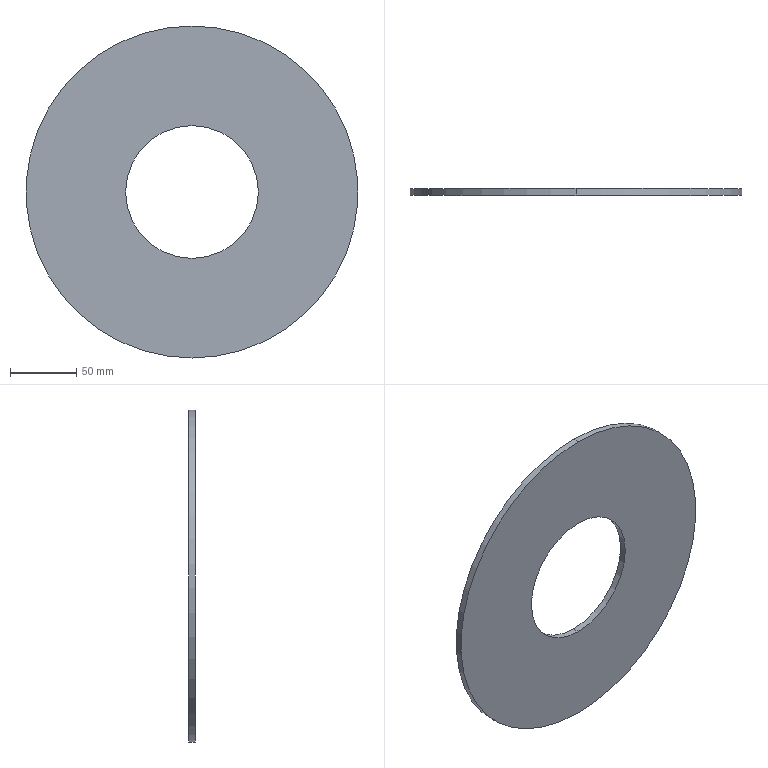Component | SolidWorks | Support2-2 | 1 solid | 6 faces | box 250 x 5 x 250 mm | volume 206167 mm3 | cylinder 4 | plane 2 | commonest cylinder face diameters 100 x2 250 x2 | material Plain Carbon Steel
STEP:
#1=COLOUR_RGB('',0.7922,0.8196,0.9333);
#2=FILL_AREA_STYLE_COLOUR('',#1);
#3=FILL_AREA_STYLE('',(#2));
#4=SURFACE_STYLE_FILL_AREA(#3);
#5=SURFACE_SIDE_STYLE('',(#4));
#6=SURFACE_STYLE_USAGE(.BOTH.,#5);
#7=PRESENTATION_STYLE_ASSIGNMENT((#6));
#8=CARTESIAN_POINT('',(49.235,57.14,70.988));
#9=VERTEX_POINT('',#8);
#10=CARTESIAN_POINT('',(49.235,57.14,74.925));
#11=VERTEX_POINT('',#10);
#12=CARTESIAN_POINT('',(49.235,57.14,72.956));
#13=DIRECTION('',(-0.,-1.,-0.));
#14=DIRECTION('',(0.,-0.,1.));
#15=AXIS2_PLACEMENT_3D('',#12,#13,#14);
#16=CIRCLE('',#15,1.969);
#17=EDGE_CURVE('',#9,#11,#16,.T.);
#18=ORIENTED_EDGE('',*,*,#17,.F.);
#19=CARTESIAN_POINT('',(49.235,56.943,70.988));
#20=VERTEX_POINT('',#19);
#21=CARTESIAN_POINT('',(49.235,57.14,70.988));
#22=DIRECTION('',(-0.,-1.,-0.));
#23=VECTOR('',#22,39.37);
#24=LINE('',#21,#23);
#25=EDGE_CURVE('',#9,#20,#24,.T.);
#26=ORIENTED_EDGE('',*,*,#25,.T.);
#27=CARTESIAN_POINT('',(49.235,56.943,74.925));
#28=VERTEX_POINT('',#27);
#29=CARTESIAN_POINT('',(49.235,56.943,72.956));
#30=DIRECTION('',(-0.,-1.,-0.));
#31=DIRECTION('',(0.,-0.,1.));
#32=AXIS2_PLACEMENT_3D('',#29,#30,#31);
#33=CIRCLE('',#32,1.969);
#34=EDGE_CURVE('',#20,#28,#33,.T.);
#35=ORIENTED_EDGE('',*,*,#34,.T.);
#36=CARTESIAN_POINT('',(49.235,57.14,74.925));
#37=DIRECTION('',(-0.,-1.,-0.));
#38=VECTOR('',#37,39.37);
#39=LINE('',#36,#38);
#40=EDGE_CURVE('',#11,#28,#39,.T.);
#41=ORIENTED_EDGE('',*,*,#40,.F.);
#42=EDGE_LOOP('',(#18,#26,#35,#41));
#43=FACE_OUTER_BOUND('',#42,.T.);
#44=CARTESIAN_POINT('',(49.235,57.14,72.956));
#45=DIRECTION('',(-0.,-1.,-0.));
#46=DIRECTION('',(0.,-0.,1.));
#47=AXIS2_PLACEMENT_3D('',#44,#45,#46);
#48=CYLINDRICAL_SURFACE('',#47,1.969);
#49=ADVANCED_FACE('',(#43),#48,.F.);
#50=CARTESIAN_POINT('',(49.235,57.14,77.877));
#51=VERTEX_POINT('',#50);
#52=CARTESIAN_POINT('',(49.235,57.14,68.035));
#53=VERTEX_POINT('',#52);
#54=CARTESIAN_POINT('',(49.235,57.14,72.956));
#55=DIRECTION('',(-0.,-1.,-0.));
#56=DIRECTION('',(0.,-0.,1.));
#57=AXIS2_PLACEMENT_3D('',#54,#55,#56);
#58=CIRCLE('',#57,4.921);
#59=EDGE_CURVE('',#51,#53,#58,.T.);
#60=ORIENTED_EDGE('',*,*,#59,.T.);
#61=CARTESIAN_POINT('',(49.235,56.943,68.035));
#62=VERTEX_POINT('',#61);
#63=CARTESIAN_POINT('',(49.235,57.14,68.035));
#64=DIRECTION('',(-0.,-1.,-0.));
#65=VECTOR('',#64,39.37);
#66=LINE('',#63,#65);
#67=EDGE_CURVE('',#53,#62,#66,.T.);
#68=ORIENTED_EDGE('',*,*,#67,.T.);
#69=CARTESIAN_POINT('',(49.235,56.943,77.877));
#70=VERTEX_POINT('',#69);
#71=CARTESIAN_POINT('',(49.235,56.943,72.956));
#72=DIRECTION('',(-0.,-1.,-0.));
#73=DIRECTION('',(0.,-0.,1.));
#74=AXIS2_PLACEMENT_3D('',#71,#72,#73);
#75=CIRCLE('',#74,4.921);
#76=EDGE_CURVE('',#70,#62,#75,.T.);
#77=ORIENTED_EDGE('',*,*,#76,.F.);
#78=CARTESIAN_POINT('',(49.235,57.14,77.877));
#79=DIRECTION('',(-0.,-1.,-0.));
#80=VECTOR('',#79,39.37);
#81=LINE('',#78,#80);
#82=EDGE_CURVE('',#51,#70,#81,.T.);
#83=ORIENTED_EDGE('',*,*,#82,.F.);
#84=EDGE_LOOP('',(#60,#68,#77,#83));
#85=FACE_OUTER_BOUND('',#84,.T.);
#86=CARTESIAN_POINT('',(49.235,57.14,72.956));
#87=DIRECTION('',(-0.,-1.,-0.));
#88=DIRECTION('',(0.,-0.,1.));
#89=AXIS2_PLACEMENT_3D('',#86,#87,#88);
#90=CYLINDRICAL_SURFACE('',#89,4.921);
#91=ADVANCED_FACE('',(#85),#90,.T.);
#92=ORIENTED_EDGE('',*,*,#67,.F.);
#93=CARTESIAN_POINT('',(49.235,57.14,72.956));
#94=DIRECTION('',(-0.,-1.,-0.));
#95=DIRECTION('',(0.,-0.,1.));
#96=AXIS2_PLACEMENT_3D('',#93,#94,#95);
#97=CIRCLE('',#96,4.921);
#98=EDGE_CURVE('',#53,#51,#97,.T.);
#99=ORIENTED_EDGE('',*,*,#98,.T.);
#100=ORIENTED_EDGE('',*,*,#82,.T.);
#101=CARTESIAN_POINT('',(49.235,56.943,72.956));
#102=DIRECTION('',(-0.,-1.,-0.));
#103=DIRECTION('',(0.,-0.,1.));
#104=AXIS2_PLACEMENT_3D('',#101,#102,#103);
#105=CIRCLE('',#104,4.921);
#106=EDGE_CURVE('',#62,#70,#105,.T.);
#107=ORIENTED_EDGE('',*,*,#106,.F.);
#108=EDGE_LOOP('',(#92,#99,#100,#107));
#109=FACE_OUTER_BOUND('',#108,.T.);
#110=CARTESIAN_POINT('',(49.235,57.14,72.956));
#111=DIRECTION('',(-0.,-1.,-0.));
#112=DIRECTION('',(0.,-0.,1.));
#113=AXIS2_PLACEMENT_3D('',#110,#111,#112);
#114=CYLINDRICAL_SURFACE('',#113,4.921);
#115=ADVANCED_FACE('',(#109),#114,.T.);
#116=CARTESIAN_POINT('',(49.235,57.14,72.956));
#117=DIRECTION('',(-0.,-1.,-0.));
#118=DIRECTION('',(0.,-0.,1.));
#119=AXIS2_PLACEMENT_3D('',#116,#117,#118);
#120=CIRCLE('',#119,1.969);
#121=EDGE_CURVE('',#11,#9,#120,.T.);
#122=ORIENTED_EDGE('',*,*,#121,.T.);
#123=ORIENTED_EDGE('',*,*,#17,.T.);
#124=EDGE_LOOP('',(#122,#123));
#125=FACE_BOUND('',#124,.T.);
#126=ORIENTED_EDGE('',*,*,#59,.F.);
#127=ORIENTED_EDGE('',*,*,#98,.F.);
#128=EDGE_LOOP('',(#126,#127));
#129=FACE_OUTER_BOUND('',#128,.T.);
#130=CARTESIAN_POINT('',(49.235,57.14,72.956));
#131=DIRECTION('',(-0.,-1.,-0.));
#132=DIRECTION('',(0.,-0.,1.));
#133=AXIS2_PLACEMENT_3D('',#130,#131,#132);
#134=PLANE('',#133);
#135=ADVANCED_FACE('',(#125,#129),#134,.F.);
#136=CARTESIAN_POINT('',(49.235,56.943,72.956));
#137=DIRECTION('',(-0.,-1.,-0.));
#138=DIRECTION('',(0.,-0.,1.));
#139=AXIS2_PLACEMENT_3D('',#136,#137,#138);
#140=CIRCLE('',#139,1.969);
#141=EDGE_CURVE('',#28,#20,#140,.T.);
#142=ORIENTED_EDGE('',*,*,#141,.F.);
#143=ORIENTED_EDGE('',*,*,#34,.F.);
#144=EDGE_LOOP('',(#142,#143));
#145=FACE_BOUND('',#144,.T.);
#146=ORIENTED_EDGE('',*,*,#76,.T.);
#147=ORIENTED_EDGE('',*,*,#106,.T.);
#148=EDGE_LOOP('',(#146,#147));
#149=FACE_OUTER_BOUND('',#148,.T.);
#150=CARTESIAN_POINT('',(49.235,56.943,72.956));
#151=DIRECTION('',(-0.,-1.,-0.));
#152=DIRECTION('',(0.,-0.,1.));
#153=AXIS2_PLACEMENT_3D('',#150,#151,#152);
#154=PLANE('',#153);
#155=ADVANCED_FACE('',(#145,#149),#154,.T.);
#156=ORIENTED_EDGE('',*,*,#25,.F.);
#157=ORIENTED_EDGE('',*,*,#121,.F.);
#158=ORIENTED_EDGE('',*,*,#40,.T.);
#159=ORIENTED_EDGE('',*,*,#141,.T.);
#160=EDGE_LOOP('',(#156,#157,#158,#159));
#161=FACE_OUTER_BOUND('',#160,.T.);
#162=CARTESIAN_POINT('',(49.235,57.14,72.956));
#163=DIRECTION('',(-0.,-1.,-0.));
#164=DIRECTION('',(0.,-0.,1.));
#165=AXIS2_PLACEMENT_3D('',#162,#163,#164);
#166=CYLINDRICAL_SURFACE('',#165,1.969);
#167=ADVANCED_FACE('',(#161),#166,.F.);
#168=CLOSED_SHELL('',(#49,#91,#115,#135,#155,#167));
#169=MANIFOLD_SOLID_BREP('',#168);
#170=STYLED_ITEM('',(#7),#169);
#171=PRESENTATION_LAYER_ASSIGNMENT('','',(#170));
#172=CARTESIAN_POINT('',(0.,0.,0.));
#173=DIRECTION('',(0.,0.,1.));
#174=DIRECTION('',(1.,0.,0.));
#175=AXIS2_PLACEMENT_3D('',#172,#173,#174);
#176=(LENGTH_UNIT()NAMED_UNIT(*)SI_UNIT($,.METRE.));
#177=LENGTH_MEASURE_WITH_UNIT(LENGTH_MEASURE(0.0254),#176);
#178=DIMENSIONAL_EXPONENTS(1.,0.,0.,0.,0.,0.,0.);
#179=(CONVERSION_BASED_UNIT('',#177)LENGTH_UNIT()NAMED_UNIT(#178));
#180=UNCERTAINTY_MEASURE_WITH_UNIT(LENGTH_MEASURE(0.00001),#179,'','');
#181=(NAMED_UNIT(*)PLANE_ANGLE_UNIT()SI_UNIT($,.RADIAN.));
#182=(NAMED_UNIT(*)SI_UNIT($,.STERADIAN.)SOLID_ANGLE_UNIT());
#183=(GEOMETRIC_REPRESENTATION_CONTEXT(3)GLOBAL_UNCERTAINTY_ASSIGNED_CONTEXT((#180))GLOBAL_UNIT_ASSIGNED_CONTEXT((#179,#181,#182))REPRESENTATION_CONTEXT('',''));
#184=ADVANCED_BREP_SHAPE_REPRESENTATION('',(#169,#175),#183);
#185=(LENGTH_UNIT()NAMED_UNIT(*)SI_UNIT($,.METRE.));
#186=LENGTH_MEASURE_WITH_UNIT(LENGTH_MEASURE(0.0254),#185);
#187=DIMENSIONAL_EXPONENTS(1.,0.,0.,0.,0.,0.,0.);
#188=(CONVERSION_BASED_UNIT('',#186)LENGTH_UNIT()NAMED_UNIT(#187));
#189=UNCERTAINTY_MEASURE_WITH_UNIT(LENGTH_MEASURE(0.00001),#188,'','');
#190=(NAMED_UNIT(*)PLANE_ANGLE_UNIT()SI_UNIT($,.RADIAN.));
#191=(NAMED_UNIT(*)SI_UNIT($,.STERADIAN.)SOLID_ANGLE_UNIT());
#192=(GEOMETRIC_REPRESENTATION_CONTEXT(3)GLOBAL_UNCERTAINTY_ASSIGNED_CONTEXT((#189))GLOBAL_UNIT_ASSIGNED_CONTEXT((#188,#190,#191))REPRESENTATION_CONTEXT('',''));
#193=MECHANICAL_DESIGN_GEOMETRIC_PRESENTATION_REPRESENTATION('',(#170),#192);